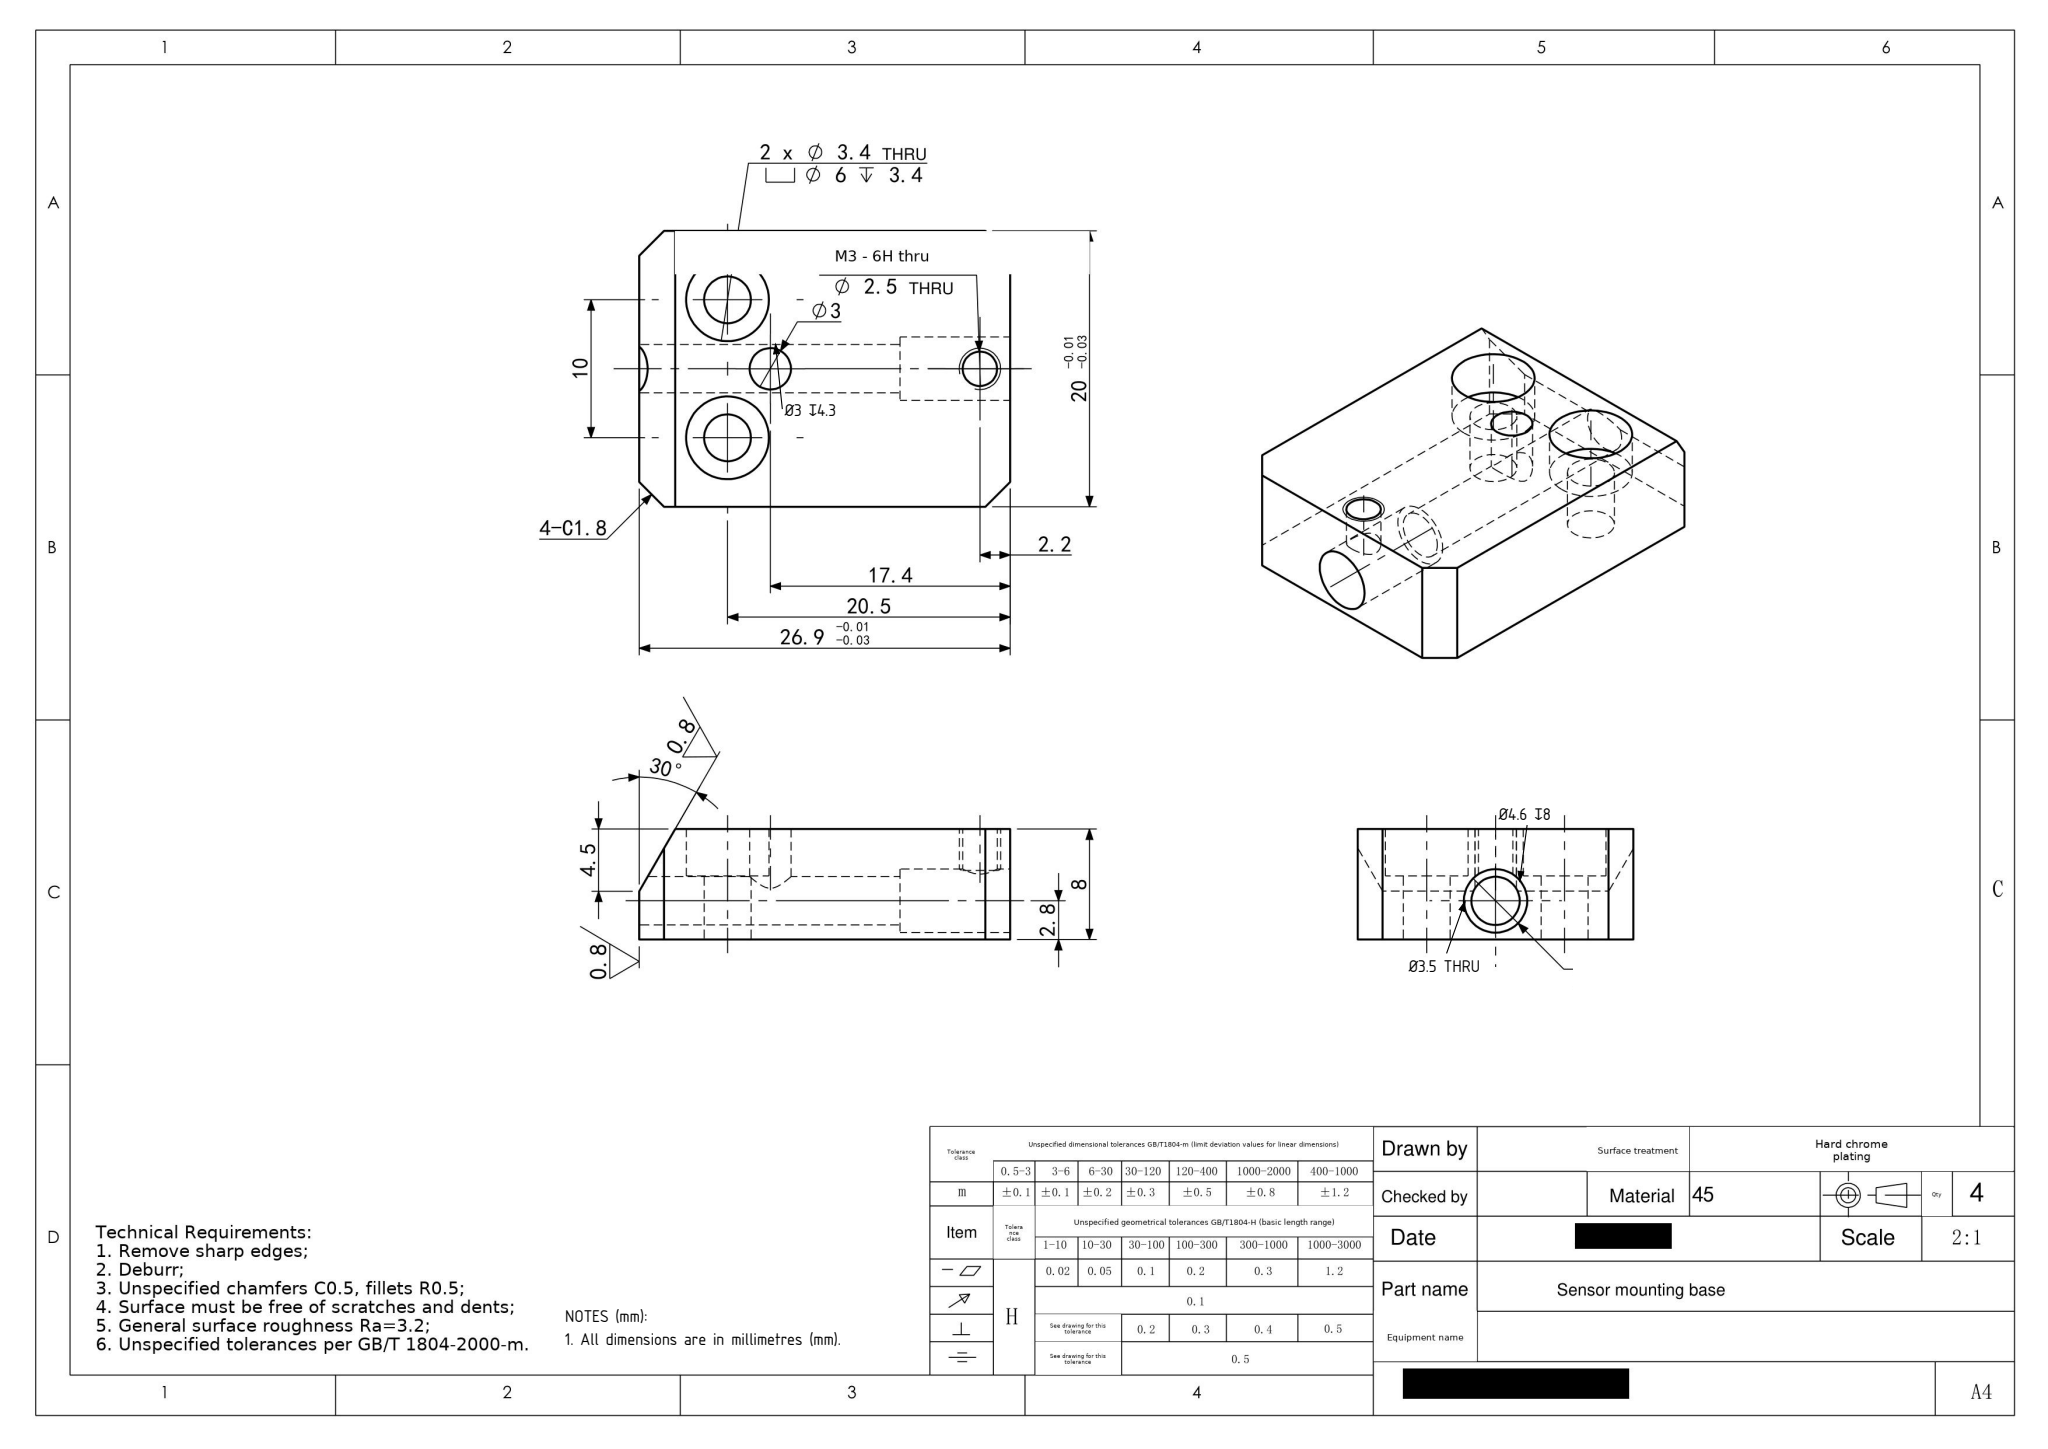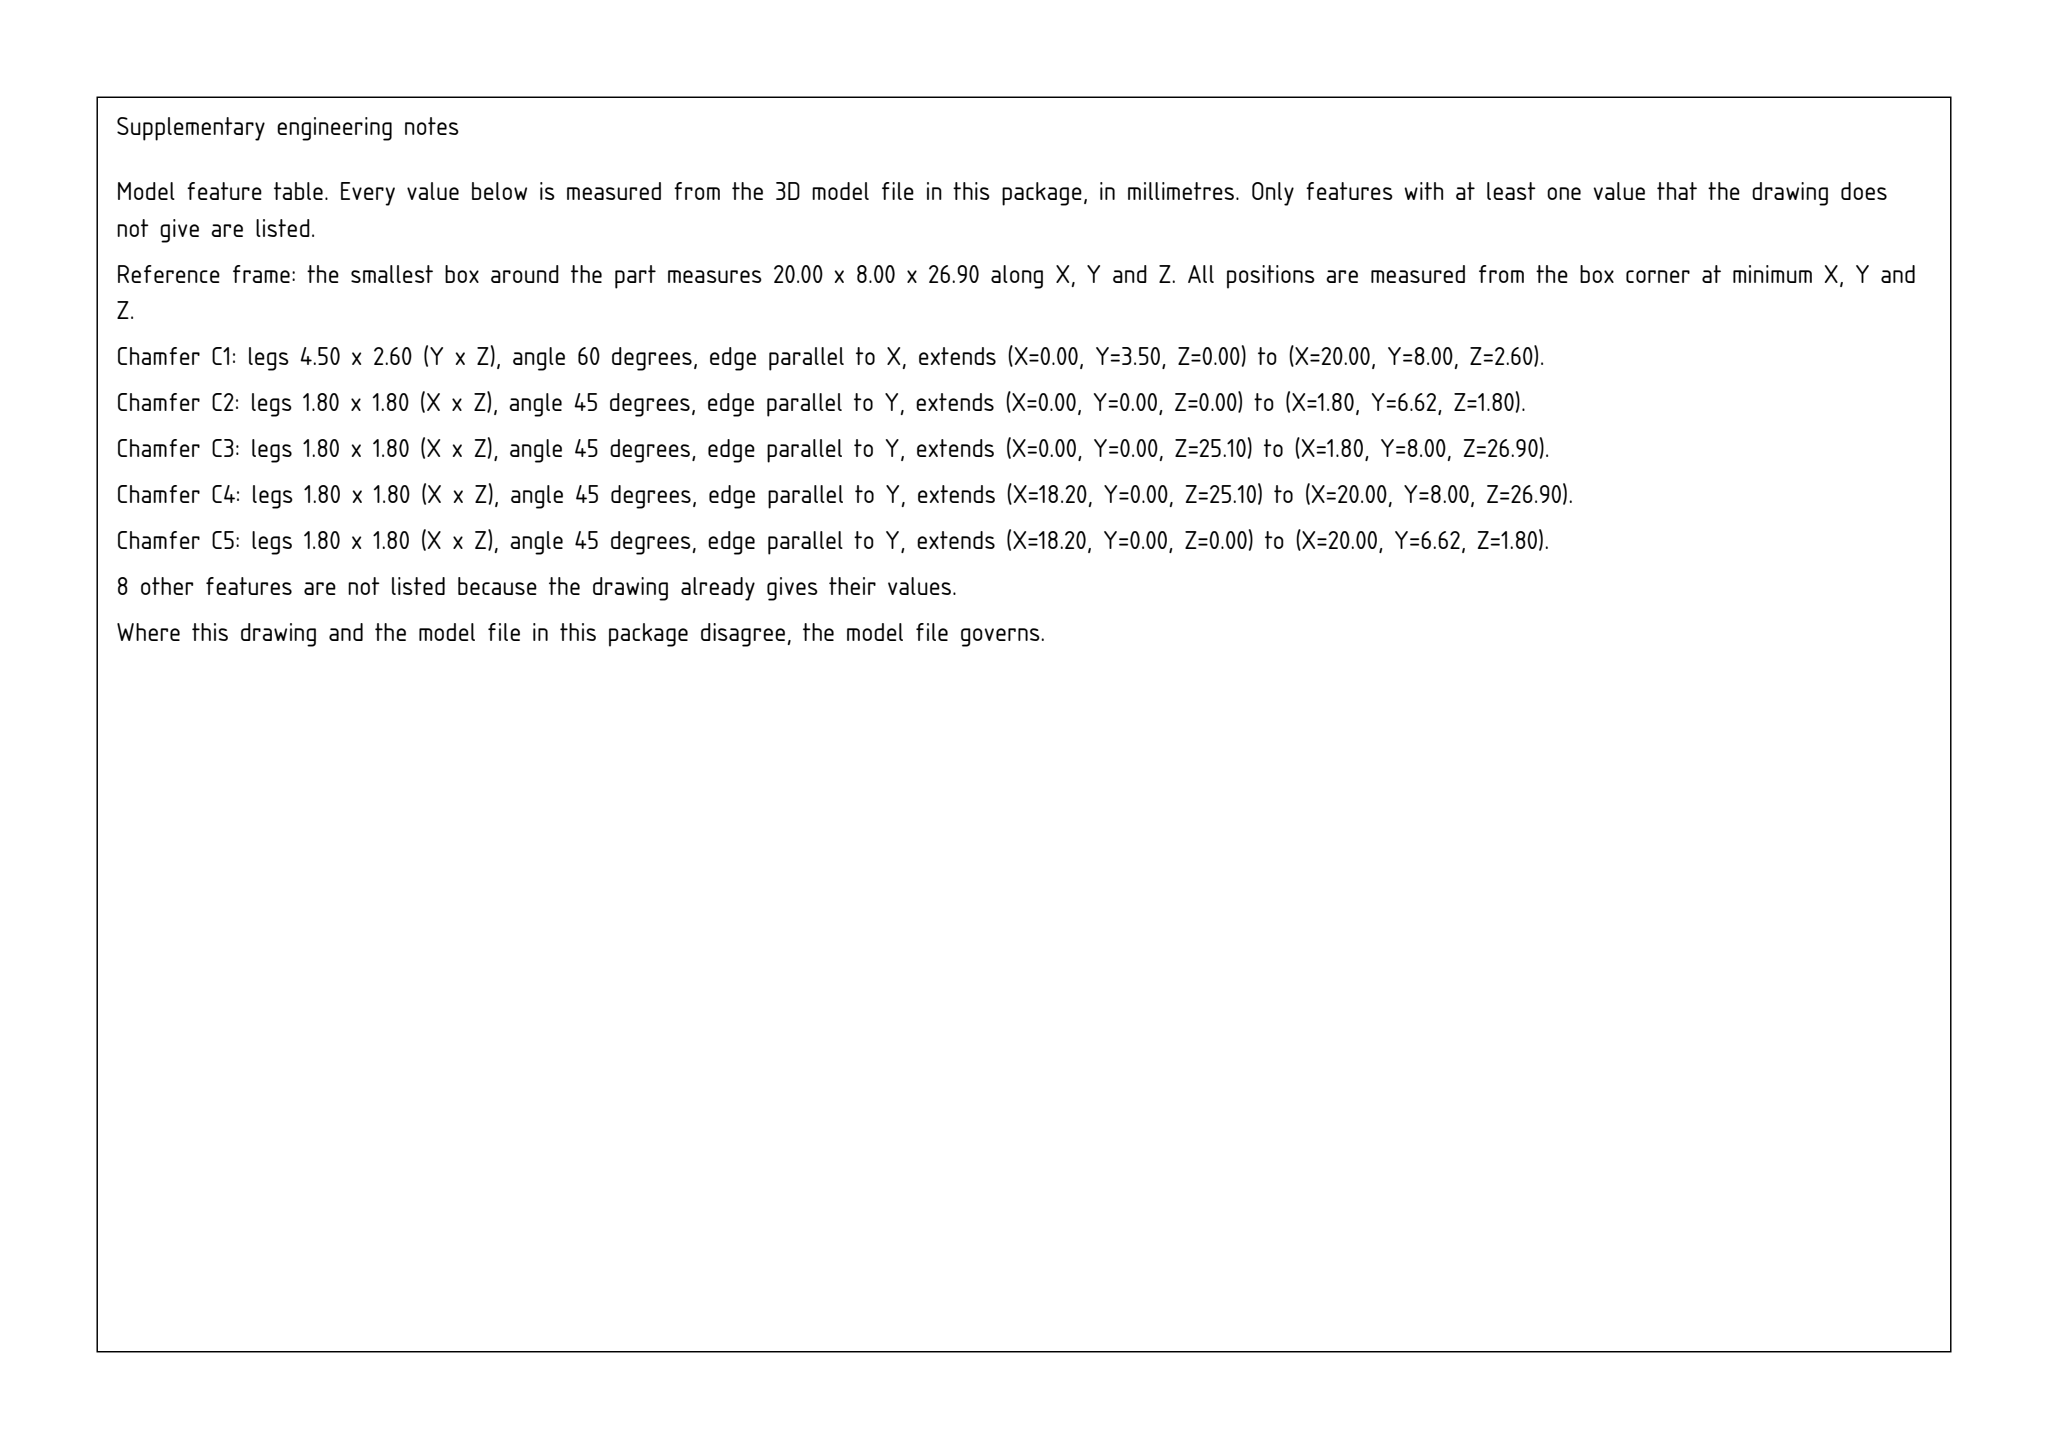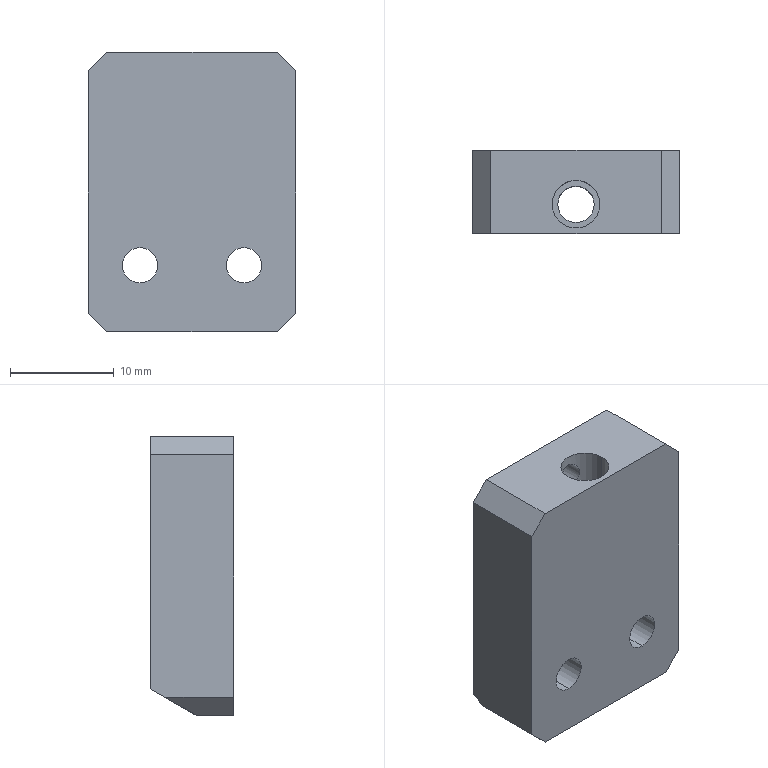Part | SolidWorks | mm | material 45 | 1 solid | 30 faces | box 20 x 8 x 26.9 mm | volume 3516 mm3 | cylinder 16 | plane 14 | commonest cylinder face diameters 6 x4 3.4 x4 3 x2 4.6 x2 2.5 x2 3.5 x2
Drawing notes:
Lengthwise bore: Ø3.5 THRU (26.9 long), axis centred 10 from each side face and 2.8 above bottom face. | from the solid: cylinders: [3.5,"z",[10.0,2.8,null],18.9] plus [4.6,"z",[10.0,2.8,null],8.0] = 26.9 total = bbox z
Counterbore for the lengthwise bore: Ø4.6 DP 8, entering from the end face at z=26.9 (the same end as the Ø2.5 THRU hole, whose axis lies 2.2 from that end face); coaxial with the Ø3.5 bore, which runs 18.9 from the opposite end face. | from the solid: cylinders: Ø4.6 axis z at (x=10, y=2.8) from z=18.9 to z=26.9; Ø3.5 axis z at (x=10, y=2.8) from z=0 to z=18.9; Ø2.5 hole axis at z=24.7 (= 2.2 from the z=26.9 end face)
Middle top hole: Ø3 blind, depth 4.3 from top face, breaking into the Ø3.5 lengthwise bore; axis 17.4 from the end face at z=26.9 and 10 from each side face. | from the solid: cylinder [3.0,"y",[10.0,null,9.5],4.3]; bbox y=8 so 8-4.3=3.7 reaching Ø3.5 bore at y=2.8
All dimensions are in millimetres (mm). | from the solid: STEP model units: mm (bbox_xyz 20.0 x 8.0 x 26.9 mm)
build123d program:
from build123d import *

# Parameters (mm, degrees)
SKETCH1_W                                       = 20
SKETCH1_H                                       = 26.9
BOSS_EXTRUDE1_DEPTH                             = 8
CUT_EXTRUDE1_REACH                              = 31.793
SKETCH2_R                                       = 1.75
M3_HEX_SOCKET_HEAD_CAP_SCREW_CBORE1_D           = 3.4
M3_HEX_SOCKET_HEAD_CAP_SCREW_CBORE1_CBORE_D     = 6
M3_HEX_SOCKET_HEAD_CAP_SCREW_CBORE1_CBORE_DEPTH = 3.4
M3_TAPPED_HOLE1_REACH                           = 20.572
M3_TAPPED_HOLE1_BORE_R                          = 1.25
CUT_EXTRUDE2_REACH                              = 27.395
CHAMFER1_SIZE                                   = 1.8
SKETCH8_R                                       = 2.3
CUT_EXTRUDE3_DEPTH                              = 8
CUT_EXTRUDE4_REACH                              = 20.572
CUT_EXTRUDE4_END_RADIUS                         = 1.75
SKETCH9_R                                       = 1.5


with BuildPart() as part:
    # Sketch1 → Boss-Extrude1 (new body)
    with BuildSketch(Plane(origin=(0, 0, 0), x_dir=(1, 0, 0), z_dir=(0, 1, 0))):
        Rectangle(SKETCH1_W, SKETCH1_H)
    extrude(amount=BOSS_EXTRUDE1_DEPTH)

    # Sketch2 → Cut-Extrude1 (cut, up to next)
    with BuildSketch(Plane.XY.offset(13.45), mode=Mode.PRIVATE) as cut_extrude1_sk1:
        with Locations((0, 2.8)):
            Circle(SKETCH2_R)
    cut_extrude1_tool1 = extrude(cut_extrude1_sk1.sketch, amount=-CUT_EXTRUDE1_REACH, mode=Mode.PRIVATE) & part.part
    add(cut_extrude1_tool1.solids().sort_by_distance((0, 2.8, 13.45))[0], mode=Mode.SUBTRACT)

    # M3 Hex Socket Head Cap Screw CBORE1 (through all)
    with Locations(Plane(origin=(0, 8, 0), x_dir=(1, 0, 0), z_dir=(0, 1, 0))):
        with Locations((-5, 7.05), (5, 7.05)):
            CounterBoreHole(M3_HEX_SOCKET_HEAD_CAP_SCREW_CBORE1_D / 2, M3_HEX_SOCKET_HEAD_CAP_SCREW_CBORE1_CBORE_D / 2, M3_HEX_SOCKET_HEAD_CAP_SCREW_CBORE1_CBORE_DEPTH)

    # M3 Tapped Hole1 bore → M3 Tapped Hole1 (cut, up to next)
    with BuildSketch(Plane(origin=(0, 8, 0), x_dir=(1, 0, 0), z_dir=(0, 1, 0)), mode=Mode.PRIVATE) as m3_tapped_hole1_sk1:
        with Locations((0, -11.25)):
            Circle(M3_TAPPED_HOLE1_BORE_R)
    m3_tapped_hole1_tool1 = extrude(m3_tapped_hole1_sk1.sketch, amount=-M3_TAPPED_HOLE1_REACH, mode=Mode.PRIVATE) & part.part
    add(m3_tapped_hole1_tool1.solids().sort_by_distance((0, 8, 11.25))[0], mode=Mode.SUBTRACT)

    # Sketch7 → Cut-Extrude2 (cut, up to next)
    with BuildSketch(Plane(origin=(10, 0, 0), x_dir=(0, 0, -1), z_dir=(1, 0, 0)), mode=Mode.PRIVATE) as cut_extrude2_sk1:
        Polygon((13.45, 3.5), (10.852, 8), (13.45, 8), align=None)
    cut_extrude2_tool1 = extrude(cut_extrude2_sk1.sketch, amount=-CUT_EXTRUDE2_REACH, mode=Mode.PRIVATE) & part.part
    add(cut_extrude2_tool1.solids().sort_by_distance((10, 6.5, -12.584))[0], mode=Mode.SUBTRACT)

    # Chamfer1
    chamfer1_edges = [part.edges().sort_by_distance(p)[0] for p in [
        (-10, 1.75, -13.45),
        (10, 1.75, -13.45),
        (10, 4, 13.45),
        (-10, 4, 13.45),
    ]]
    chamfer(chamfer1_edges, length=CHAMFER1_SIZE)

    # Sketch8 → Cut-Extrude3 (cut)
    with BuildSketch(Plane.XY.offset(13.45)):
        with Locations((0, 2.8)):
            Circle(SKETCH8_R)
    extrude(amount=-CUT_EXTRUDE3_DEPTH, mode=Mode.SUBTRACT)

    # Cut-Extrude4: up to this cylinder (the profile starts outside it)
    cut_extrude4_end = Plane(origin=(0, 2.8, -3.95), z_dir=(0, 0, 1)) * Cylinder(CUT_EXTRUDE4_END_RADIUS, 45.644, mode=Mode.PRIVATE)
    # Sketch9 → Cut-Extrude4 (cut, up to the surface)
    with BuildSketch(Plane(origin=(0, 8, 0), x_dir=(1, 0, 0), z_dir=(0, 1, 0)), mode=Mode.PRIVATE) as cut_extrude4_sk1:
        with Locations(Location((0, 3.95, 0), (0, 0, 270))):
            Circle(SKETCH9_R)
    cut_extrude4_tool1 = extrude(cut_extrude4_sk1.sketch, amount=-CUT_EXTRUDE4_REACH, mode=Mode.PRIVATE) - cut_extrude4_end
    add(cut_extrude4_tool1.solids().sort_by_distance((0, 8, -3.95))[0], mode=Mode.SUBTRACT)


solid = part.part